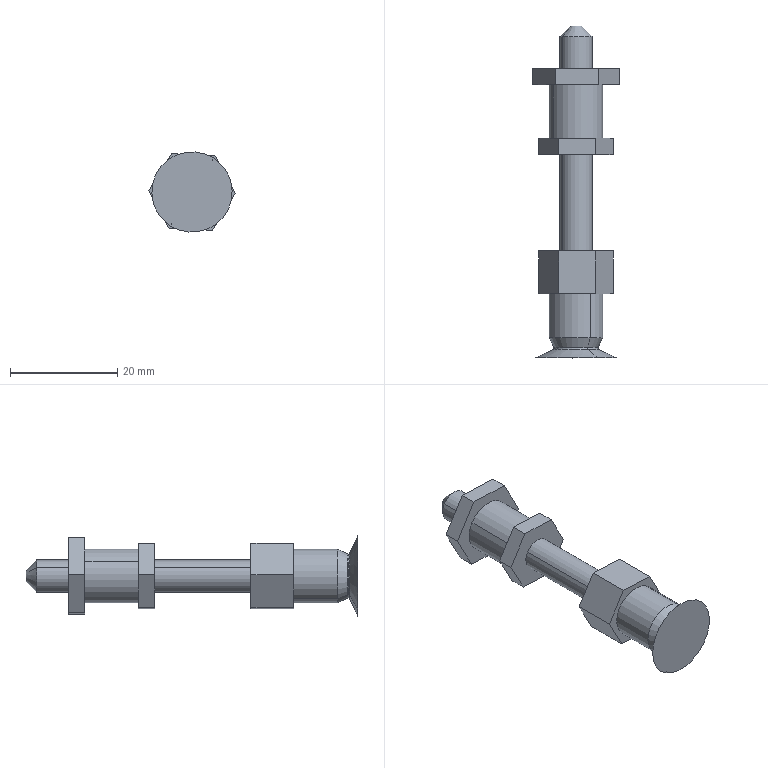Component | SolidWorks | SL021-1SuctionCup.SL4PRT-1 | 1 solid | 44 faces | volume 4329 mm3 | plane 26 | cylinder 8 | cone 6 | torus 4 | commonest cylinder face diameters 10 x4 6 x4 | material AL6061